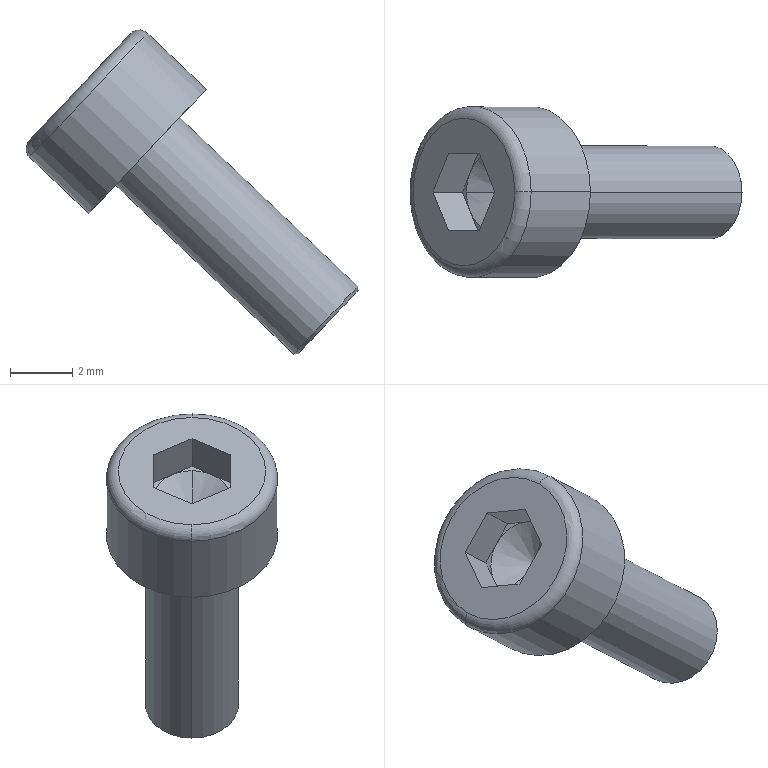Component | SolidWorks | 100-1_hexagon socket head cap screws gb_GB_FASTENER_SCREWS_HSHCS M3X8-N-1 | 1 solid | 25 faces | box 10.68 x 5.5 x 10.43 mm | volume 119 mm3 | plane 15 | cone 4 | cylinder 4 | torus 2 | commonest cylinder face diameters 3 x2 5.5 x2
STEP:
#1=COLOUR_RGB('',0.7922,0.8196,0.9333);
#2=FILL_AREA_STYLE_COLOUR('',#1);
#3=FILL_AREA_STYLE('',(#2));
#4=SURFACE_STYLE_FILL_AREA(#3);
#5=SURFACE_SIDE_STYLE('',(#4));
#6=SURFACE_STYLE_USAGE(.BOTH.,#5);
#7=PRESENTATION_STYLE_ASSIGNMENT((#6));
#8=CARTESIAN_POINT('',(20.6,49.134,-79.959));
#9=VERTEX_POINT('',#8);
#10=CARTESIAN_POINT('',(20.6,49.134,-79.954));
#11=VERTEX_POINT('',#10);
#12=CARTESIAN_POINT('',(20.6,49.134,-79.959));
#13=DIRECTION('',(-0.02683,-0.,0.9996));
#14=VECTOR('',#13,39.37);
#15=LINE('',#12,#14);
#16=EDGE_CURVE('',#9,#11,#15,.T.);
#17=ORIENTED_EDGE('',*,*,#16,.F.);
#18=CARTESIAN_POINT('',(20.524,49.134,-80.039));
#19=VERTEX_POINT('',#18);
#20=CARTESIAN_POINT('',(20.562,49.134,-79.999));
#21=DIRECTION('',(0.7258,0.,-0.6879));
#22=DIRECTION('',(0.6879,-0.,0.7258));
#23=AXIS2_PLACEMENT_3D('',#20,#21,#22);
#24=CIRCLE('',#23,0.05512);
#25=EDGE_CURVE('',#19,#9,#24,.T.);
#26=ORIENTED_EDGE('',*,*,#25,.F.);
#27=CARTESIAN_POINT('',(20.518,49.134,-80.039));
#28=VERTEX_POINT('',#27);
#29=CARTESIAN_POINT('',(20.524,49.134,-80.039));
#30=DIRECTION('',(-0.9996,0.,-0.02683));
#31=VECTOR('',#30,39.37);
#32=LINE('',#29,#31);
#33=EDGE_CURVE('',#19,#28,#32,.T.);
#34=ORIENTED_EDGE('',*,*,#33,.T.);
#35=CARTESIAN_POINT('',(20.559,49.134,-79.997));
#36=DIRECTION('',(-0.7258,-0.,0.6879));
#37=DIRECTION('',(0.6879,-0.,0.7258));
#38=AXIS2_PLACEMENT_3D('',#35,#36,#37);
#39=CIRCLE('',#38,0.05906);
#40=EDGE_CURVE('',#11,#28,#39,.T.);
#41=ORIENTED_EDGE('',*,*,#40,.F.);
#42=EDGE_LOOP('',(#17,#26,#34,#41));
#43=FACE_OUTER_BOUND('',#42,.T.);
#44=CARTESIAN_POINT('',(20.562,49.134,-79.999));
#45=DIRECTION('',(-0.7258,-0.,0.6879));
#46=DIRECTION('',(-0.6879,0.,-0.7258));
#47=AXIS2_PLACEMENT_3D('',#44,#45,#46);
#48=CONICAL_SURFACE('',#47,0.05512,0.7854);
#49=ADVANCED_FACE('',(#43),#48,.T.);
#50=CARTESIAN_POINT('',(20.183,49.134,-79.769));
#51=VERTEX_POINT('',#50);
#52=CARTESIAN_POINT('',(20.184,49.134,-79.79));
#53=VERTEX_POINT('',#52);
#54=CARTESIAN_POINT('',(20.194,49.134,-79.779));
#55=DIRECTION('',(-0.,-1.,-0.));
#56=DIRECTION('',(-0.6879,0.,-0.7258));
#57=AXIS2_PLACEMENT_3D('',#54,#55,#56);
#58=CIRCLE('',#57,0.01476);
#59=EDGE_CURVE('',#51,#53,#58,.T.);
#60=ORIENTED_EDGE('',*,*,#59,.F.);
#61=CARTESIAN_POINT('',(20.312,49.134,-79.633));
#62=VERTEX_POINT('',#61);
#63=CARTESIAN_POINT('',(20.248,49.134,-79.701));
#64=DIRECTION('',(-0.7258,-0.,0.6879));
#65=DIRECTION('',(0.6879,-0.,0.7258));
#66=AXIS2_PLACEMENT_3D('',#63,#64,#65);
#67=CIRCLE('',#66,0.0935);
#68=EDGE_CURVE('',#62,#51,#67,.T.);
#69=ORIENTED_EDGE('',*,*,#68,.F.);
#70=CARTESIAN_POINT('',(20.333,49.134,-79.633));
#71=VERTEX_POINT('',#70);
#72=CARTESIAN_POINT('',(20.323,49.134,-79.644));
#73=DIRECTION('',(0.,1.,0.));
#74=DIRECTION('',(0.6879,0.,0.7258));
#75=AXIS2_PLACEMENT_3D('',#72,#73,#74);
#76=CIRCLE('',#75,0.01476);
#77=EDGE_CURVE('',#62,#71,#76,.T.);
#78=ORIENTED_EDGE('',*,*,#77,.T.);
#79=CARTESIAN_POINT('',(20.258,49.134,-79.712));
#80=DIRECTION('',(0.7258,0.,-0.6879));
#81=DIRECTION('',(0.6879,-0.,0.7258));
#82=AXIS2_PLACEMENT_3D('',#79,#80,#81);
#83=CIRCLE('',#82,0.1083);
#84=EDGE_CURVE('',#53,#71,#83,.T.);
#85=ORIENTED_EDGE('',*,*,#84,.F.);
#86=EDGE_LOOP('',(#60,#69,#78,#85));
#87=FACE_OUTER_BOUND('',#86,.T.);
#88=CARTESIAN_POINT('',(20.258,49.134,-79.712));
#89=DIRECTION('',(0.7258,0.,-0.6879));
#90=DIRECTION('',(0.6879,-0.,0.7258));
#91=AXIS2_PLACEMENT_3D('',#88,#89,#90);
#92=TOROIDAL_SURFACE('',#91,0.0935,0.01476);
#93=ADVANCED_FACE('',(#87),#92,.T.);
#94=CARTESIAN_POINT('',(20.305,49.134,-79.756));
#95=VERTEX_POINT('',#94);
#96=CARTESIAN_POINT('',(20.319,49.134,-79.701));
#97=VERTEX_POINT('',#96);
#98=CARTESIAN_POINT('',(20.319,49.134,-79.701));
#99=DIRECTION('',(0.2328,-0.,0.9725));
#100=VECTOR('',#99,39.37);
#101=LINE('',#98,#100);
#102=EDGE_CURVE('',#95,#97,#101,.T.);
#103=ORIENTED_EDGE('',*,*,#102,.F.);
#104=CARTESIAN_POINT('',(20.251,49.134,-79.772));
#105=VERTEX_POINT('',#104);
#106=CARTESIAN_POINT('',(20.251,49.134,-79.772));
#107=DIRECTION('',(-0.9586,0.,-0.2846));
#108=VECTOR('',#107,39.37);
#109=LINE('',#106,#108);
#110=EDGE_CURVE('',#95,#105,#109,.T.);
#111=ORIENTED_EDGE('',*,*,#110,.T.);
#112=CARTESIAN_POINT('',(20.255,49.109,-79.767));
#113=VERTEX_POINT('',#112);
#114=CARTESIAN_POINT('',(20.285,49.134,-79.737));
#115=DIRECTION('',(-0.7258,-0.,0.6879));
#116=DIRECTION('',(0.6879,-0.,0.7258));
#117=AXIS2_PLACEMENT_3D('',#114,#115,#116);
#118=CIRCLE('',#117,0.04921);
#119=EDGE_CURVE('',#105,#113,#118,.T.);
#120=ORIENTED_EDGE('',*,*,#119,.T.);
#121=CARTESIAN_POINT('',(20.285,49.085,-79.737));
#122=VERTEX_POINT('',#121);
#123=CARTESIAN_POINT('',(20.285,49.134,-79.737));
#124=DIRECTION('',(-0.7258,-0.,0.6879));
#125=DIRECTION('',(0.6879,-0.,0.7258));
#126=AXIS2_PLACEMENT_3D('',#123,#124,#125);
#127=CIRCLE('',#126,0.04921);
#128=EDGE_CURVE('',#113,#122,#127,.T.);
#129=ORIENTED_EDGE('',*,*,#128,.T.);
#130=CARTESIAN_POINT('',(20.314,49.109,-79.706));
#131=VERTEX_POINT('',#130);
#132=CARTESIAN_POINT('',(20.285,49.134,-79.737));
#133=DIRECTION('',(0.7258,0.,-0.6879));
#134=DIRECTION('',(0.6879,-0.,0.7258));
#135=AXIS2_PLACEMENT_3D('',#132,#133,#134);
#136=CIRCLE('',#135,0.04921);
#137=EDGE_CURVE('',#131,#122,#136,.T.);
#138=ORIENTED_EDGE('',*,*,#137,.F.);
#139=CARTESIAN_POINT('',(20.285,49.134,-79.737));
#140=DIRECTION('',(-0.7258,-0.,0.6879));
#141=DIRECTION('',(0.6879,-0.,0.7258));
#142=AXIS2_PLACEMENT_3D('',#139,#140,#141);
#143=CIRCLE('',#142,0.04921);
#144=EDGE_CURVE('',#131,#97,#143,.T.);
#145=ORIENTED_EDGE('',*,*,#144,.T.);
#146=EDGE_LOOP('',(#103,#111,#120,#129,#138,#145));
#147=FACE_OUTER_BOUND('',#146,.T.);
#148=CARTESIAN_POINT('',(20.285,49.134,-79.737));
#149=DIRECTION('',(-0.7258,-0.,0.6879));
#150=DIRECTION('',(-0.6879,0.,-0.7258));
#151=AXIS2_PLACEMENT_3D('',#148,#149,#150);
#152=CONICAL_SURFACE('',#151,0.04921,1.047);
#153=ADVANCED_FACE('',(#147),#152,.F.);
#154=CARTESIAN_POINT('',(20.228,49.183,-79.722));
#155=VERTEX_POINT('',#154);
#156=CARTESIAN_POINT('',(20.267,49.183,-79.681));
#157=VERTEX_POINT('',#156);
#158=CARTESIAN_POINT('',(20.228,49.183,-79.722));
#159=DIRECTION('',(0.6879,-0.,0.7258));
#160=VECTOR('',#159,39.37);
#161=LINE('',#158,#160);
#162=EDGE_CURVE('',#155,#157,#161,.T.);
#163=ORIENTED_EDGE('',*,*,#162,.F.);
#164=CARTESIAN_POINT('',(20.265,49.183,-79.757));
#165=VERTEX_POINT('',#164);
#166=CARTESIAN_POINT('',(20.265,49.183,-79.757));
#167=DIRECTION('',(-0.7258,-0.,0.6879));
#168=VECTOR('',#167,39.37);
#169=LINE('',#166,#168);
#170=EDGE_CURVE('',#165,#155,#169,.T.);
#171=ORIENTED_EDGE('',*,*,#170,.F.);
#172=CARTESIAN_POINT('',(20.285,49.183,-79.737));
#173=VERTEX_POINT('',#172);
#174=CARTESIAN_POINT('',(20.265,49.183,-79.757));
#175=DIRECTION('',(0.6879,-0.,0.7258));
#176=VECTOR('',#175,39.37);
#177=LINE('',#174,#176);
#178=EDGE_CURVE('',#165,#173,#177,.T.);
#179=ORIENTED_EDGE('',*,*,#178,.T.);
#180=CARTESIAN_POINT('',(20.304,49.183,-79.716));
#181=VERTEX_POINT('',#180);
#182=CARTESIAN_POINT('',(20.265,49.183,-79.757));
#183=DIRECTION('',(0.6879,-0.,0.7258));
#184=VECTOR('',#183,39.37);
#185=LINE('',#182,#184);
#186=EDGE_CURVE('',#173,#181,#185,.T.);
#187=ORIENTED_EDGE('',*,*,#186,.T.);
#188=CARTESIAN_POINT('',(20.304,49.183,-79.716));
#189=DIRECTION('',(-0.7258,-0.,0.6879));
#190=VECTOR('',#189,39.37);
#191=LINE('',#188,#190);
#192=EDGE_CURVE('',#181,#157,#191,.T.);
#193=ORIENTED_EDGE('',*,*,#192,.T.);
#194=EDGE_LOOP('',(#163,#171,#179,#187,#193));
#195=FACE_OUTER_BOUND('',#194,.T.);
#196=CARTESIAN_POINT('',(20.265,49.183,-79.757));
#197=DIRECTION('',(-0.,-1.,-0.));
#198=DIRECTION('',(0.7258,0.,-0.6879));
#199=AXIS2_PLACEMENT_3D('',#196,#197,#198);
#200=PLANE('',#199);
#201=ADVANCED_FACE('',(#195),#200,.T.);
#202=CARTESIAN_POINT('',(20.209,49.134,-79.743));
#203=VERTEX_POINT('',#202);
#204=CARTESIAN_POINT('',(20.209,49.134,-79.743));
#205=DIRECTION('',(0.3439,0.866,0.3629));
#206=VECTOR('',#205,39.37);
#207=LINE('',#204,#206);
#208=EDGE_CURVE('',#203,#155,#207,.T.);
#209=ORIENTED_EDGE('',*,*,#208,.F.);
#210=CARTESIAN_POINT('',(20.246,49.134,-79.778));
#211=VERTEX_POINT('',#210);
#212=CARTESIAN_POINT('',(20.246,49.134,-79.778));
#213=DIRECTION('',(-0.7258,-0.,0.6879));
#214=VECTOR('',#213,39.37);
#215=LINE('',#212,#214);
#216=EDGE_CURVE('',#211,#203,#215,.T.);
#217=ORIENTED_EDGE('',*,*,#216,.F.);
#218=CARTESIAN_POINT('',(20.255,49.158,-79.767));
#219=VERTEX_POINT('',#218);
#220=CARTESIAN_POINT('',(20.246,49.134,-79.778));
#221=DIRECTION('',(0.3439,0.866,0.3629));
#222=VECTOR('',#221,39.37);
#223=LINE('',#220,#222);
#224=EDGE_CURVE('',#211,#219,#223,.T.);
#225=ORIENTED_EDGE('',*,*,#224,.T.);
#226=CARTESIAN_POINT('',(20.246,49.134,-79.778));
#227=DIRECTION('',(0.3439,0.866,0.3629));
#228=VECTOR('',#227,39.37);
#229=LINE('',#226,#228);
#230=EDGE_CURVE('',#219,#165,#229,.T.);
#231=ORIENTED_EDGE('',*,*,#230,.T.);
#232=ORIENTED_EDGE('',*,*,#170,.T.);
#233=EDGE_LOOP('',(#209,#217,#225,#231,#232));
#234=FACE_OUTER_BOUND('',#233,.T.);
#235=CARTESIAN_POINT('',(20.246,49.134,-79.778));
#236=DIRECTION('',(0.5957,-0.5,0.6286));
#237=DIRECTION('',(-0.7258,-0.,0.6879));
#238=AXIS2_PLACEMENT_3D('',#235,#236,#237);
#239=PLANE('',#238);
#240=ADVANCED_FACE('',(#234),#239,.T.);
#241=CARTESIAN_POINT('',(20.228,49.085,-79.722));
#242=VERTEX_POINT('',#241);
#243=CARTESIAN_POINT('',(20.228,49.085,-79.722));
#244=DIRECTION('',(-0.3439,0.866,-0.3629));
#245=VECTOR('',#244,39.37);
#246=LINE('',#243,#245);
#247=EDGE_CURVE('',#242,#203,#246,.T.);
#248=ORIENTED_EDGE('',*,*,#247,.F.);
#249=CARTESIAN_POINT('',(20.265,49.085,-79.757));
#250=VERTEX_POINT('',#249);
#251=CARTESIAN_POINT('',(20.265,49.085,-79.757));
#252=DIRECTION('',(-0.7258,-0.,0.6879));
#253=VECTOR('',#252,39.37);
#254=LINE('',#251,#253);
#255=EDGE_CURVE('',#250,#242,#254,.T.);
#256=ORIENTED_EDGE('',*,*,#255,.F.);
#257=CARTESIAN_POINT('',(20.265,49.085,-79.757));
#258=DIRECTION('',(-0.3439,0.866,-0.3629));
#259=VECTOR('',#258,39.37);
#260=LINE('',#257,#259);
#261=EDGE_CURVE('',#250,#113,#260,.T.);
#262=ORIENTED_EDGE('',*,*,#261,.T.);
#263=CARTESIAN_POINT('',(20.265,49.085,-79.757));
#264=DIRECTION('',(-0.3439,0.866,-0.3629));
#265=VECTOR('',#264,39.37);
#266=LINE('',#263,#265);
#267=EDGE_CURVE('',#113,#211,#266,.T.);
#268=ORIENTED_EDGE('',*,*,#267,.T.);
#269=ORIENTED_EDGE('',*,*,#216,.T.);
#270=EDGE_LOOP('',(#248,#256,#262,#268,#269));
#271=FACE_OUTER_BOUND('',#270,.T.);
#272=CARTESIAN_POINT('',(20.265,49.085,-79.757));
#273=DIRECTION('',(0.5957,0.5,0.6286));
#274=DIRECTION('',(-0.3439,0.866,-0.3629));
#275=AXIS2_PLACEMENT_3D('',#272,#273,#274);
#276=PLANE('',#275);
#277=ADVANCED_FACE('',(#271),#276,.T.);
#278=CARTESIAN_POINT('',(20.267,49.085,-79.681));
#279=VERTEX_POINT('',#278);
#280=CARTESIAN_POINT('',(20.267,49.085,-79.681));
#281=DIRECTION('',(-0.6879,0.,-0.7258));
#282=VECTOR('',#281,39.37);
#283=LINE('',#280,#282);
#284=EDGE_CURVE('',#279,#242,#283,.T.);
#285=ORIENTED_EDGE('',*,*,#284,.F.);
#286=CARTESIAN_POINT('',(20.304,49.085,-79.716));
#287=VERTEX_POINT('',#286);
#288=CARTESIAN_POINT('',(20.304,49.085,-79.716));
#289=DIRECTION('',(-0.7258,-0.,0.6879));
#290=VECTOR('',#289,39.37);
#291=LINE('',#288,#290);
#292=EDGE_CURVE('',#287,#279,#291,.T.);
#293=ORIENTED_EDGE('',*,*,#292,.F.);
#294=CARTESIAN_POINT('',(20.304,49.085,-79.716));
#295=DIRECTION('',(-0.6879,0.,-0.7258));
#296=VECTOR('',#295,39.37);
#297=LINE('',#294,#296);
#298=EDGE_CURVE('',#287,#122,#297,.T.);
#299=ORIENTED_EDGE('',*,*,#298,.T.);
#300=CARTESIAN_POINT('',(20.304,49.085,-79.716));
#301=DIRECTION('',(-0.6879,0.,-0.7258));
#302=VECTOR('',#301,39.37);
#303=LINE('',#300,#302);
#304=EDGE_CURVE('',#122,#250,#303,.T.);
#305=ORIENTED_EDGE('',*,*,#304,.T.);
#306=ORIENTED_EDGE('',*,*,#255,.T.);
#307=EDGE_LOOP('',(#285,#293,#299,#305,#306));
#308=FACE_OUTER_BOUND('',#307,.T.);
#309=CARTESIAN_POINT('',(20.304,49.085,-79.716));
#310=DIRECTION('',(0.,1.,0.));
#311=DIRECTION('',(0.6879,-0.,0.7258));
#312=AXIS2_PLACEMENT_3D('',#309,#310,#311);
#313=PLANE('',#312);
#314=ADVANCED_FACE('',(#308),#313,.T.);
#315=CARTESIAN_POINT('',(20.287,49.134,-79.66));
#316=VERTEX_POINT('',#315);
#317=CARTESIAN_POINT('',(20.287,49.134,-79.66));
#318=DIRECTION('',(-0.3439,-0.866,-0.3629));
#319=VECTOR('',#318,39.37);
#320=LINE('',#317,#319);
#321=EDGE_CURVE('',#316,#279,#320,.T.);
#322=ORIENTED_EDGE('',*,*,#321,.F.);
#323=CARTESIAN_POINT('',(20.324,49.134,-79.695));
#324=VERTEX_POINT('',#323);
#325=CARTESIAN_POINT('',(20.324,49.134,-79.695));
#326=DIRECTION('',(-0.7258,-0.,0.6879));
#327=VECTOR('',#326,39.37);
#328=LINE('',#325,#327);
#329=EDGE_CURVE('',#324,#316,#328,.T.);
#330=ORIENTED_EDGE('',*,*,#329,.F.);
#331=CARTESIAN_POINT('',(20.324,49.134,-79.695));
#332=DIRECTION('',(-0.3439,-0.866,-0.3629));
#333=VECTOR('',#332,39.37);
#334=LINE('',#331,#333);
#335=EDGE_CURVE('',#324,#131,#334,.T.);
#336=ORIENTED_EDGE('',*,*,#335,.T.);
#337=CARTESIAN_POINT('',(20.324,49.134,-79.695));
#338=DIRECTION('',(-0.3439,-0.866,-0.3629));
#339=VECTOR('',#338,39.37);
#340=LINE('',#337,#339);
#341=EDGE_CURVE('',#131,#287,#340,.T.);
#342=ORIENTED_EDGE('',*,*,#341,.T.);
#343=ORIENTED_EDGE('',*,*,#292,.T.);
#344=EDGE_LOOP('',(#322,#330,#336,#342,#343));
#345=FACE_OUTER_BOUND('',#344,.T.);
#346=CARTESIAN_POINT('',(20.324,49.134,-79.695));
#347=DIRECTION('',(-0.5957,0.5,-0.6286));
#348=DIRECTION('',(-0.7258,-0.,0.6879));
#349=AXIS2_PLACEMENT_3D('',#346,#347,#348);
#350=PLANE('',#349);
#351=ADVANCED_FACE('',(#345),#350,.T.);
#352=CARTESIAN_POINT('',(20.267,49.183,-79.681));
#353=DIRECTION('',(0.3439,-0.866,0.3629));
#354=VECTOR('',#353,39.37);
#355=LINE('',#352,#354);
#356=EDGE_CURVE('',#157,#316,#355,.T.);
#357=ORIENTED_EDGE('',*,*,#356,.F.);
#358=ORIENTED_EDGE('',*,*,#192,.F.);
#359=CARTESIAN_POINT('',(20.314,49.158,-79.706));
#360=VERTEX_POINT('',#359);
#361=CARTESIAN_POINT('',(20.304,49.183,-79.716));
#362=DIRECTION('',(0.3439,-0.866,0.3629));
#363=VECTOR('',#362,39.37);
#364=LINE('',#361,#363);
#365=EDGE_CURVE('',#181,#360,#364,.T.);
#366=ORIENTED_EDGE('',*,*,#365,.T.);
#367=CARTESIAN_POINT('',(20.304,49.183,-79.716));
#368=DIRECTION('',(0.3439,-0.866,0.3629));
#369=VECTOR('',#368,39.37);
#370=LINE('',#367,#369);
#371=EDGE_CURVE('',#360,#324,#370,.T.);
#372=ORIENTED_EDGE('',*,*,#371,.T.);
#373=ORIENTED_EDGE('',*,*,#329,.T.);
#374=EDGE_LOOP('',(#357,#358,#366,#372,#373));
#375=FACE_OUTER_BOUND('',#374,.T.);
#376=CARTESIAN_POINT('',(20.304,49.183,-79.716));
#377=DIRECTION('',(-0.5957,-0.5,-0.6286));
#378=DIRECTION('',(0.7258,0.,-0.6879));
#379=AXIS2_PLACEMENT_3D('',#376,#377,#378);
#380=PLANE('',#379);
#381=ADVANCED_FACE('',(#375),#380,.T.);
#382=ORIENTED_EDGE('',*,*,#25,.T.);
#383=CARTESIAN_POINT('',(20.562,49.134,-79.999));
#384=DIRECTION('',(0.7258,0.,-0.6879));
#385=DIRECTION('',(0.6879,-0.,0.7258));
#386=AXIS2_PLACEMENT_3D('',#383,#384,#385);
#387=CIRCLE('',#386,0.05512);
#388=EDGE_CURVE('',#9,#19,#387,.T.);
#389=ORIENTED_EDGE('',*,*,#388,.T.);
#390=EDGE_LOOP('',(#382,#389));
#391=FACE_OUTER_BOUND('',#390,.T.);
#392=CARTESIAN_POINT('',(20.562,49.134,-79.999));
#393=DIRECTION('',(0.7258,0.,-0.6879));
#394=DIRECTION('',(-0.,-1.,-0.));
#395=AXIS2_PLACEMENT_3D('',#392,#393,#394);
#396=PLANE('',#395);
#397=ADVANCED_FACE('',(#391),#396,.T.);
#398=CARTESIAN_POINT('',(20.374,49.134,-79.74));
#399=VERTEX_POINT('',#398);
#400=CARTESIAN_POINT('',(20.603,49.134,-79.956));
#401=DIRECTION('',(-0.7258,-0.,0.6879));
#402=VECTOR('',#401,39.37);
#403=LINE('',#400,#402);
#404=EDGE_CURVE('',#11,#399,#403,.T.);
#405=ORIENTED_EDGE('',*,*,#404,.F.);
#406=ORIENTED_EDGE('',*,*,#40,.T.);
#407=CARTESIAN_POINT('',(20.293,49.134,-79.825));
#408=VERTEX_POINT('',#407);
#409=CARTESIAN_POINT('',(20.521,49.134,-80.042));
#410=DIRECTION('',(-0.7258,-0.,0.6879));
#411=VECTOR('',#410,39.37);
#412=LINE('',#409,#411);
#413=EDGE_CURVE('',#28,#408,#412,.T.);
#414=ORIENTED_EDGE('',*,*,#413,.T.);
#415=CARTESIAN_POINT('',(20.333,49.134,-79.783));
#416=DIRECTION('',(0.7258,0.,-0.6879));
#417=DIRECTION('',(0.6879,-0.,0.7258));
#418=AXIS2_PLACEMENT_3D('',#415,#416,#417);
#419=CIRCLE('',#418,0.05906);
#420=EDGE_CURVE('',#408,#399,#419,.T.);
#421=ORIENTED_EDGE('',*,*,#420,.T.);
#422=EDGE_LOOP('',(#405,#406,#414,#421));
#423=FACE_OUTER_BOUND('',#422,.T.);
#424=CARTESIAN_POINT('',(20.562,49.134,-79.999));
#425=DIRECTION('',(-0.7258,-0.,0.6879));
#426=DIRECTION('',(-0.6879,0.,-0.7258));
#427=AXIS2_PLACEMENT_3D('',#424,#425,#426);
#428=CYLINDRICAL_SURFACE('',#427,0.05906);
#429=ADVANCED_FACE('',(#423),#428,.T.);
#430=CARTESIAN_POINT('',(20.408,49.134,-79.704));
#431=VERTEX_POINT('',#430);
#432=CARTESIAN_POINT('',(20.408,49.134,-79.704));
#433=DIRECTION('',(-0.7258,-0.,0.6879));
#434=VECTOR('',#433,39.37);
#435=LINE('',#432,#434);
#436=EDGE_CURVE('',#431,#71,#435,.T.);
#437=ORIENTED_EDGE('',*,*,#436,.F.);
#438=CARTESIAN_POINT('',(20.259,49.134,-79.861));
#439=VERTEX_POINT('',#438);
#440=CARTESIAN_POINT('',(20.333,49.134,-79.783));
#441=DIRECTION('',(0.7258,0.,-0.6879));
#442=DIRECTION('',(0.6879,-0.,0.7258));
#443=AXIS2_PLACEMENT_3D('',#440,#441,#442);
#444=CIRCLE('',#443,0.1083);
#445=EDGE_CURVE('',#439,#431,#444,.T.);
#446=ORIENTED_EDGE('',*,*,#445,.F.);
#447=CARTESIAN_POINT('',(20.259,49.134,-79.861));
#448=DIRECTION('',(-0.7258,-0.,0.6879));
#449=VECTOR('',#448,39.37);
#450=LINE('',#447,#449);
#451=EDGE_CURVE('',#439,#53,#450,.T.);
#452=ORIENTED_EDGE('',*,*,#451,.T.);
#453=ORIENTED_EDGE('',*,*,#84,.T.);
#454=EDGE_LOOP('',(#437,#446,#452,#453));
#455=FACE_OUTER_BOUND('',#454,.T.);
#456=CARTESIAN_POINT('',(20.333,49.134,-79.783));
#457=DIRECTION('',(-0.7258,-0.,0.6879));
#458=DIRECTION('',(-0.6879,0.,-0.7258));
#459=AXIS2_PLACEMENT_3D('',#456,#457,#458);
#460=CYLINDRICAL_SURFACE('',#459,0.1083);
#461=ADVANCED_FACE('',(#455),#460,.T.);
#462=ORIENTED_EDGE('',*,*,#420,.F.);
#463=CARTESIAN_POINT('',(20.333,49.134,-79.783));
#464=DIRECTION('',(0.7258,0.,-0.6879));
#465=DIRECTION('',(0.6879,-0.,0.7258));
#466=AXIS2_PLACEMENT_3D('',#463,#464,#465);
#467=CIRCLE('',#466,0.05906);
#468=EDGE_CURVE('',#399,#408,#467,.T.);
#469=ORIENTED_EDGE('',*,*,#468,.F.);
#470=EDGE_LOOP('',(#462,#469));
#471=FACE_BOUND('',#470,.T.);
#472=ORIENTED_EDGE('',*,*,#445,.T.);
#473=CARTESIAN_POINT('',(20.333,49.134,-79.783));
#474=DIRECTION('',(0.7258,0.,-0.6879));
#475=DIRECTION('',(0.6879,-0.,0.7258));
#476=AXIS2_PLACEMENT_3D('',#473,#474,#475);
#477=CIRCLE('',#476,0.1083);
#478=EDGE_CURVE('',#431,#439,#477,.T.);
#479=ORIENTED_EDGE('',*,*,#478,.T.);
#480=EDGE_LOOP('',(#472,#479));
#481=FACE_OUTER_BOUND('',#480,.T.);
#482=CARTESIAN_POINT('',(20.333,49.134,-79.783));
#483=DIRECTION('',(0.7258,0.,-0.6879));
#484=DIRECTION('',(-0.,-1.,-0.));
#485=AXIS2_PLACEMENT_3D('',#482,#483,#484);
#486=PLANE('',#485);
#487=ADVANCED_FACE('',(#471,#481),#486,.T.);
#488=ORIENTED_EDGE('',*,*,#356,.T.);
#489=ORIENTED_EDGE('',*,*,#321,.T.);
#490=ORIENTED_EDGE('',*,*,#284,.T.);
#491=ORIENTED_EDGE('',*,*,#247,.T.);
#492=ORIENTED_EDGE('',*,*,#208,.T.);
#493=ORIENTED_EDGE('',*,*,#162,.T.);
#494=EDGE_LOOP('',(#488,#489,#490,#491,#492,#493));
#495=FACE_BOUND('',#494,.T.);
#496=ORIENTED_EDGE('',*,*,#68,.T.);
#497=CARTESIAN_POINT('',(20.248,49.134,-79.701));
#498=DIRECTION('',(-0.7258,-0.,0.6879));
#499=DIRECTION('',(0.6879,-0.,0.7258));
#500=AXIS2_PLACEMENT_3D('',#497,#498,#499);
#501=CIRCLE('',#500,0.0935);
#502=EDGE_CURVE('',#51,#62,#501,.T.);
#503=ORIENTED_EDGE('',*,*,#502,.T.);
#504=EDGE_LOOP('',(#496,#503));
#505=FACE_OUTER_BOUND('',#504,.T.);
#506=CARTESIAN_POINT('',(20.248,49.134,-79.701));
#507=DIRECTION('',(0.7258,0.,-0.6879));
#508=DIRECTION('',(-0.,-1.,-0.));
#509=AXIS2_PLACEMENT_3D('',#506,#507,#508);
#510=PLANE('',#509);
#511=ADVANCED_FACE('',(#495,#505),#510,.F.);
#512=ORIENTED_EDGE('',*,*,#144,.F.);
#513=ORIENTED_EDGE('',*,*,#335,.F.);
#514=ORIENTED_EDGE('',*,*,#371,.F.);
#515=CARTESIAN_POINT('',(20.285,49.134,-79.737));
#516=DIRECTION('',(-0.7258,-0.,0.6879));
#517=DIRECTION('',(0.6879,-0.,0.7258));
#518=AXIS2_PLACEMENT_3D('',#515,#516,#517);
#519=CIRCLE('',#518,0.04921);
#520=EDGE_CURVE('',#97,#360,#519,.T.);
#521=ORIENTED_EDGE('',*,*,#520,.F.);
#522=EDGE_LOOP('',(#512,#513,#514,#521));
#523=FACE_OUTER_BOUND('',#522,.T.);
#524=CARTESIAN_POINT('',(20.324,49.134,-79.695));
#525=DIRECTION('',(0.7258,0.,-0.6879));
#526=DIRECTION('',(-0.,-1.,-0.));
#527=AXIS2_PLACEMENT_3D('',#524,#525,#526);
#528=PLANE('',#527);
#529=ADVANCED_FACE('',(#523),#528,.F.);
#530=ORIENTED_EDGE('',*,*,#137,.T.);
#531=ORIENTED_EDGE('',*,*,#298,.F.);
#532=ORIENTED_EDGE('',*,*,#341,.F.);
#533=EDGE_LOOP('',(#530,#531,#532));
#534=FACE_OUTER_BOUND('',#533,.T.);
#535=CARTESIAN_POINT('',(20.324,49.134,-79.695));
#536=DIRECTION('',(0.7258,0.,-0.6879));
#537=DIRECTION('',(-0.,-1.,-0.));
#538=AXIS2_PLACEMENT_3D('',#535,#536,#537);
#539=PLANE('',#538);
#540=ADVANCED_FACE('',(#534),#539,.F.);
#541=ORIENTED_EDGE('',*,*,#128,.F.);
#542=ORIENTED_EDGE('',*,*,#261,.F.);
#543=ORIENTED_EDGE('',*,*,#304,.F.);
#544=EDGE_LOOP('',(#541,#542,#543));
#545=FACE_OUTER_BOUND('',#544,.T.);
#546=CARTESIAN_POINT('',(20.324,49.134,-79.695));
#547=DIRECTION('',(0.7258,0.,-0.6879));
#548=DIRECTION('',(-0.,-1.,-0.));
#549=AXIS2_PLACEMENT_3D('',#546,#547,#548);
#550=PLANE('',#549);
#551=ADVANCED_FACE('',(#545),#550,.F.);
#552=CARTESIAN_POINT('',(20.285,49.134,-79.737));
#553=DIRECTION('',(-0.7258,-0.,0.6879));
#554=DIRECTION('',(0.6879,-0.,0.7258));
#555=AXIS2_PLACEMENT_3D('',#552,#553,#554);
#556=CIRCLE('',#555,0.04921);
#557=EDGE_CURVE('',#219,#105,#556,.T.);
#558=ORIENTED_EDGE('',*,*,#557,.F.);
#559=ORIENTED_EDGE('',*,*,#224,.F.);
#560=ORIENTED_EDGE('',*,*,#267,.F.);
#561=ORIENTED_EDGE('',*,*,#119,.F.);
#562=EDGE_LOOP('',(#558,#559,#560,#561));
#563=FACE_OUTER_BOUND('',#562,.T.);
#564=CARTESIAN_POINT('',(20.324,49.134,-79.695));
#565=DIRECTION('',(0.7258,0.,-0.6879));
#566=DIRECTION('',(-0.,-1.,-0.));
#567=AXIS2_PLACEMENT_3D('',#564,#565,#566);
#568=PLANE('',#567);
#569=ADVANCED_FACE('',(#563),#568,.F.);
#570=CARTESIAN_POINT('',(20.285,49.134,-79.737));
#571=DIRECTION('',(-0.7258,-0.,0.6879));
#572=DIRECTION('',(0.6879,-0.,0.7258));
#573=AXIS2_PLACEMENT_3D('',#570,#571,#572);
#574=CIRCLE('',#573,0.04921);
#575=EDGE_CURVE('',#173,#219,#574,.T.);
#576=ORIENTED_EDGE('',*,*,#575,.F.);
#577=ORIENTED_EDGE('',*,*,#178,.F.);
#578=ORIENTED_EDGE('',*,*,#230,.F.);
#579=EDGE_LOOP('',(#576,#577,#578));
#580=FACE_OUTER_BOUND('',#579,.T.);
#581=CARTESIAN_POINT('',(20.324,49.134,-79.695));
#582=DIRECTION('',(0.7258,0.,-0.6879));
#583=DIRECTION('',(-0.,-1.,-0.));
#584=AXIS2_PLACEMENT_3D('',#581,#582,#583);
#585=PLANE('',#584);
#586=ADVANCED_FACE('',(#580),#585,.F.);
#587=CARTESIAN_POINT('',(20.285,49.134,-79.737));
#588=DIRECTION('',(-0.7258,-0.,0.6879));
#589=DIRECTION('',(0.6879,-0.,0.7258));
#590=AXIS2_PLACEMENT_3D('',#587,#588,#589);
#591=CIRCLE('',#590,0.04921);
#592=EDGE_CURVE('',#360,#173,#591,.T.);
#593=ORIENTED_EDGE('',*,*,#592,.F.);
#594=ORIENTED_EDGE('',*,*,#365,.F.);
#595=ORIENTED_EDGE('',*,*,#186,.F.);
#596=EDGE_LOOP('',(#593,#594,#595));
#597=FACE_OUTER_BOUND('',#596,.T.);
#598=CARTESIAN_POINT('',(20.324,49.134,-79.695));
#599=DIRECTION('',(0.7258,0.,-0.6879));
#600=DIRECTION('',(-0.,-1.,-0.));
#601=AXIS2_PLACEMENT_3D('',#598,#599,#600);
#602=PLANE('',#601);
#603=ADVANCED_FACE('',(#597),#602,.F.);
#604=ORIENTED_EDGE('',*,*,#478,.F.);
#605=ORIENTED_EDGE('',*,*,#436,.T.);
#606=CARTESIAN_POINT('',(20.258,49.134,-79.712));
#607=DIRECTION('',(0.7258,0.,-0.6879));
#608=DIRECTION('',(0.6879,-0.,0.7258));
#609=AXIS2_PLACEMENT_3D('',#606,#607,#608);
#610=CIRCLE('',#609,0.1083);
#611=EDGE_CURVE('',#71,#53,#610,.T.);
#612=ORIENTED_EDGE('',*,*,#611,.T.);
#613=ORIENTED_EDGE('',*,*,#451,.F.);
#614=EDGE_LOOP('',(#604,#605,#612,#613));
#615=FACE_OUTER_BOUND('',#614,.T.);
#616=CARTESIAN_POINT('',(20.333,49.134,-79.783));
#617=DIRECTION('',(-0.7258,-0.,0.6879));
#618=DIRECTION('',(-0.6879,0.,-0.7258));
#619=AXIS2_PLACEMENT_3D('',#616,#617,#618);
#620=CYLINDRICAL_SURFACE('',#619,0.1083);
#621=ADVANCED_FACE('',(#615),#620,.T.);
#622=CARTESIAN_POINT('',(20.559,49.134,-79.997));
#623=DIRECTION('',(-0.7258,-0.,0.6879));
#624=DIRECTION('',(0.6879,-0.,0.7258));
#625=AXIS2_PLACEMENT_3D('',#622,#623,#624);
#626=CIRCLE('',#625,0.05906);
#627=EDGE_CURVE('',#28,#11,#626,.T.);
#628=ORIENTED_EDGE('',*,*,#627,.T.);
#629=ORIENTED_EDGE('',*,*,#404,.T.);
#630=ORIENTED_EDGE('',*,*,#468,.T.);
#631=ORIENTED_EDGE('',*,*,#413,.F.);
#632=EDGE_LOOP('',(#628,#629,#630,#631));
#633=FACE_OUTER_BOUND('',#632,.T.);
#634=CARTESIAN_POINT('',(20.562,49.134,-79.999));
#635=DIRECTION('',(-0.7258,-0.,0.6879));
#636=DIRECTION('',(-0.6879,0.,-0.7258));
#637=AXIS2_PLACEMENT_3D('',#634,#635,#636);
#638=CYLINDRICAL_SURFACE('',#637,0.05906);
#639=ADVANCED_FACE('',(#633),#638,.T.);
#640=ORIENTED_EDGE('',*,*,#110,.F.);
#641=ORIENTED_EDGE('',*,*,#102,.T.);
#642=ORIENTED_EDGE('',*,*,#520,.T.);
#643=ORIENTED_EDGE('',*,*,#592,.T.);
#644=ORIENTED_EDGE('',*,*,#575,.T.);
#645=ORIENTED_EDGE('',*,*,#557,.T.);
#646=EDGE_LOOP('',(#640,#641,#642,#643,#644,#645));
#647=FACE_OUTER_BOUND('',#646,.T.);
#648=CARTESIAN_POINT('',(20.285,49.134,-79.737));
#649=DIRECTION('',(-0.7258,-0.,0.6879));
#650=DIRECTION('',(-0.6879,0.,-0.7258));
#651=AXIS2_PLACEMENT_3D('',#648,#649,#650);
#652=CONICAL_SURFACE('',#651,0.04921,1.047);
#653=ADVANCED_FACE('',(#647),#652,.F.);
#654=ORIENTED_EDGE('',*,*,#502,.F.);
#655=ORIENTED_EDGE('',*,*,#59,.T.);
#656=ORIENTED_EDGE('',*,*,#611,.F.);
#657=ORIENTED_EDGE('',*,*,#77,.F.);
#658=EDGE_LOOP('',(#654,#655,#656,#657));
#659=FACE_OUTER_BOUND('',#658,.T.);
#660=CARTESIAN_POINT('',(20.258,49.134,-79.712));
#661=DIRECTION('',(0.7258,0.,-0.6879));
#662=DIRECTION('',(0.6879,-0.,0.7258));
#663=AXIS2_PLACEMENT_3D('',#660,#661,#662);
#664=TOROIDAL_SURFACE('',#663,0.0935,0.01476);
#665=ADVANCED_FACE('',(#659),#664,.T.);
#666=ORIENTED_EDGE('',*,*,#388,.F.);
#667=ORIENTED_EDGE('',*,*,#16,.T.);
#668=ORIENTED_EDGE('',*,*,#627,.F.);
#669=ORIENTED_EDGE('',*,*,#33,.F.);
#670=EDGE_LOOP('',(#666,#667,#668,#669));
#671=FACE_OUTER_BOUND('',#670,.T.);
#672=CARTESIAN_POINT('',(20.562,49.134,-79.999));
#673=DIRECTION('',(-0.7258,-0.,0.6879));
#674=DIRECTION('',(-0.6879,0.,-0.7258));
#675=AXIS2_PLACEMENT_3D('',#672,#673,#674);
#676=CONICAL_SURFACE('',#675,0.05512,0.7854);
#677=ADVANCED_FACE('',(#671),#676,.T.);
#678=CLOSED_SHELL('',(#49,#93,#153,#201,#240,#277,#314,#351,#381,#397,#429,#461,#487,#511,#529,#540,#551,#569,#586,#603,#621,#639,#653,#665,#677));
#679=MANIFOLD_SOLID_BREP('',#678);
#680=STYLED_ITEM('',(#7),#679);
#681=(LENGTH_UNIT()NAMED_UNIT(*)SI_UNIT($,.METRE.));
#682=LENGTH_MEASURE_WITH_UNIT(LENGTH_MEASURE(0.0254),#681);
#683=DIMENSIONAL_EXPONENTS(1.,0.,0.,0.,0.,0.,0.);
#684=(CONVERSION_BASED_UNIT('',#682)LENGTH_UNIT()NAMED_UNIT(#683));
#685=UNCERTAINTY_MEASURE_WITH_UNIT(LENGTH_MEASURE(0.00001),#684,'','');
#686=(NAMED_UNIT(*)PLANE_ANGLE_UNIT()SI_UNIT($,.RADIAN.));
#687=(NAMED_UNIT(*)SI_UNIT($,.STERADIAN.)SOLID_ANGLE_UNIT());
#688=(GEOMETRIC_REPRESENTATION_CONTEXT(3)GLOBAL_UNCERTAINTY_ASSIGNED_CONTEXT((#685))GLOBAL_UNIT_ASSIGNED_CONTEXT((#684,#686,#687))REPRESENTATION_CONTEXT('',''));
#689=MECHANICAL_DESIGN_GEOMETRIC_PRESENTATION_REPRESENTATION('',(#680),#688);
#690=PRESENTATION_LAYER_ASSIGNMENT('','',(#680));
#691=CARTESIAN_POINT('',(0.,0.,0.));
#692=DIRECTION('',(0.,0.,1.));
#693=DIRECTION('',(1.,0.,0.));
#694=AXIS2_PLACEMENT_3D('',#691,#692,#693);
#695=(LENGTH_UNIT()NAMED_UNIT(*)SI_UNIT($,.METRE.));
#696=LENGTH_MEASURE_WITH_UNIT(LENGTH_MEASURE(0.0254),#695);
#697=DIMENSIONAL_EXPONENTS(1.,0.,0.,0.,0.,0.,0.);
#698=(CONVERSION_BASED_UNIT('',#696)LENGTH_UNIT()NAMED_UNIT(#697));
#699=UNCERTAINTY_MEASURE_WITH_UNIT(LENGTH_MEASURE(0.00001),#698,'','');
#700=(NAMED_UNIT(*)PLANE_ANGLE_UNIT()SI_UNIT($,.RADIAN.));
#701=(NAMED_UNIT(*)SI_UNIT($,.STERADIAN.)SOLID_ANGLE_UNIT());
#702=(GEOMETRIC_REPRESENTATION_CONTEXT(3)GLOBAL_UNCERTAINTY_ASSIGNED_CONTEXT((#699))GLOBAL_UNIT_ASSIGNED_CONTEXT((#698,#700,#701))REPRESENTATION_CONTEXT('',''));
#703=ADVANCED_BREP_SHAPE_REPRESENTATION('',(#679,#694),#702);